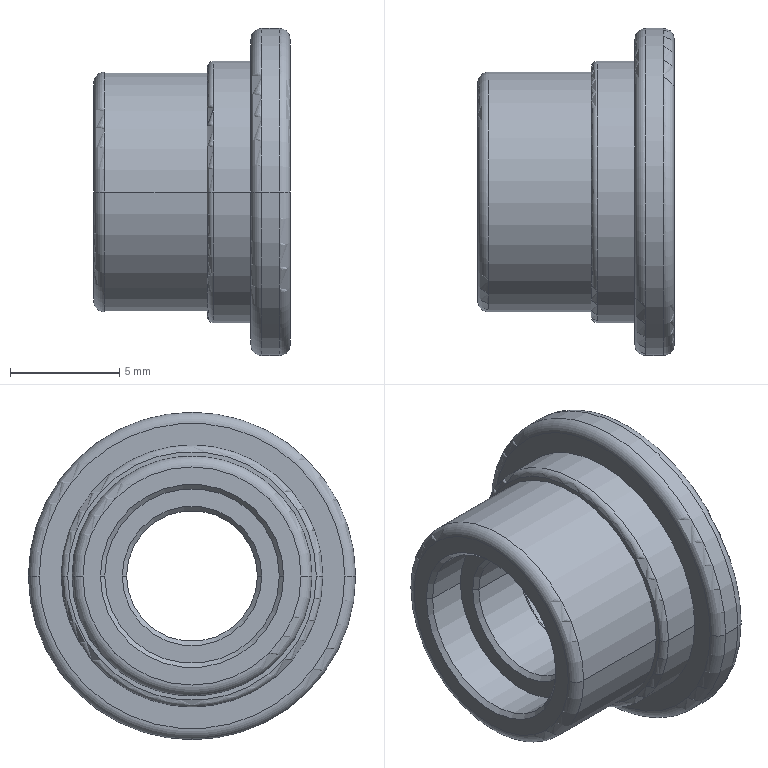Component | SolidWorks | 18MTOSC80BatteryCellCornerFoldingRollerAssembly-1_18ZTJ-NVT-01-001-1 | 1 solid | 39 faces | box 9 x 15 x 15 mm | volume 586 mm3 | cylinder 14 | cone 10 | torus 8 | plane 7 | commonest cylinder face diameters 8 x4 10 x2 11 x2 12 x2 15 x2 6 x2 | material Black POM
build123d program:
from build123d import *

# Parameters (mm, degrees)
SKETCH2_R          = 3
CUT_EXTRUDE1_DEPTH = 14.91
SKETCH3_R          = 5
CUT_EXTRUDE2_DEPTH = 2
FILLET1_R          = 0.5
FILLET2_R          = 0.3
SKETCH4_R          = 4
CUT_EXTRUDE3_DEPTH = 2
CUT_EXTRUDE4_START = -2
SKETCH5_R          = 4
CUT_EXTRUDE4_DEPTH = 2
CHAMFER1_SIZE      = 0.2


with BuildPart() as part:
    # Sketch1 → Revolve1 (revolve)
    with BuildSketch(Plane(origin=(0, 0, 0), x_dir=(1, 0, 0), z_dir=(0, 1, 0)), mode=Mode.PRIVATE) as revolve1_sk:
        Polygon((0, 0), (0, -9), (5.5, -9), (5.5, -3.8), (6, -3.8), (6, -1.8), (7.5, -1.8), (7.5, 0), align=None)
    revolve(revolve1_sk.sketch.rotate(Axis((0, 0, 0), (0, 0, 1)), 180), axis=Axis((0, 0, 0), (0, 0, 1)))

    # Sketch2 → Cut-Extrude1 (cut, through all)
    with BuildSketch(Plane.XY.offset(9)):
        Circle(SKETCH2_R)
    extrude(amount=-CUT_EXTRUDE1_DEPTH, mode=Mode.SUBTRACT)

    # Sketch3 → Cut-Extrude2 (cut)
    with BuildSketch(Plane(origin=(0, 0, 0), x_dir=(-1, 0, 0), z_dir=(0, 0, -1))):
        Circle(SKETCH3_R)
    extrude(amount=-CUT_EXTRUDE2_DEPTH, mode=Mode.SUBTRACT)

    # Fillet1
    fillet1_edges = [part.edges().sort_by_distance(p)[0] for p in [
        (5.5, 0, 9),
        (7.5, 0, 1.8),
        (7.5, 0, 0),
    ]]
    fillet(fillet1_edges, radius=FILLET1_R)

    # Fillet2
    fillet2_edges = [part.edges().sort_by_distance(p)[0] for p in [
        (6, 0, 3.8),
    ]]
    fillet(fillet2_edges, radius=FILLET2_R)

    # Sketch4 → Cut-Extrude3 (cut)
    with BuildSketch(Plane(origin=(0, 0, 2), x_dir=(-1, 0, 0), z_dir=(0, 0, -1))):
        Circle(SKETCH4_R)
    extrude(amount=-CUT_EXTRUDE3_DEPTH, mode=Mode.SUBTRACT)

    # Sketch5 → Cut-Extrude4 (cut)
    with BuildSketch(Plane.XY.offset(9).offset(CUT_EXTRUDE4_START)):
        with Locations(Location((0, 0, 0), (0, 0, 180))):
            Circle(SKETCH5_R)
    extrude(amount=CUT_EXTRUDE4_DEPTH, mode=Mode.SUBTRACT)

    # Chamfer1
    chamfer1_edges = [part.edges().sort_by_distance(p)[0] for p in [
        (5, 0, 0),
        (4, 0, 2),
        (-3, 0, 4),
        (4, 0, 9),
        (-3, 0, 7),
    ]]
    chamfer(chamfer1_edges, length=CHAMFER1_SIZE)


solid = part.part

# Placed as in the assembly
solid = solid.moved(Location((16.9, -14.53, 131), (0, -90, 0)))
STEP:
#1=CARTESIAN_POINT('',(0.6575,-0.3752,5.157));
#2=VERTEX_POINT('',#1);
#3=CARTESIAN_POINT('',(0.6575,-0.7689,5.157));
#4=VERTEX_POINT('',#3);
#5=CARTESIAN_POINT('',(0.6575,-0.572,5.157));
#6=DIRECTION('',(1.,0.,0.));
#7=DIRECTION('',(0.,1.,0.));
#8=AXIS2_PLACEMENT_3D('',#5,#6,#7);
#9=CIRCLE('',#8,0.1969);
#10=EDGE_CURVE('',#2,#4,#9,.T.);
#11=ORIENTED_EDGE('',*,*,#10,.F.);
#12=CARTESIAN_POINT('',(0.6654,-0.3673,5.157));
#13=VERTEX_POINT('',#12);
#14=CARTESIAN_POINT('',(0.6575,-0.3752,5.157));
#15=DIRECTION('',(0.7071,0.7071,-0.));
#16=VECTOR('',#15,39.37);
#17=LINE('',#14,#16);
#18=EDGE_CURVE('',#2,#13,#17,.T.);
#19=ORIENTED_EDGE('',*,*,#18,.T.);
#20=CARTESIAN_POINT('',(0.6654,-0.7768,5.157));
#21=VERTEX_POINT('',#20);
#22=CARTESIAN_POINT('',(0.6654,-0.572,5.157));
#23=DIRECTION('',(-1.,-0.,-0.));
#24=DIRECTION('',(0.,1.,0.));
#25=AXIS2_PLACEMENT_3D('',#22,#23,#24);
#26=CIRCLE('',#25,0.2047);
#27=EDGE_CURVE('',#21,#13,#26,.T.);
#28=ORIENTED_EDGE('',*,*,#27,.F.);
#29=CARTESIAN_POINT('',(0.6575,-0.7689,5.157));
#30=DIRECTION('',(0.7071,-0.7071,0.));
#31=VECTOR('',#30,39.37);
#32=LINE('',#29,#31);
#33=EDGE_CURVE('',#4,#21,#32,.T.);
#34=ORIENTED_EDGE('',*,*,#33,.F.);
#35=EDGE_LOOP('',(#11,#19,#28,#34));
#36=FACE_OUTER_BOUND('',#35,.T.);
#37=CARTESIAN_POINT('',(0.6575,-0.572,5.157));
#38=DIRECTION('',(1.,0.,0.));
#39=DIRECTION('',(0.,-1.,0.));
#40=AXIS2_PLACEMENT_3D('',#37,#38,#39);
#41=CONICAL_SURFACE('',#40,0.1969,0.7854);
#42=ADVANCED_FACE('',(#36),#41,.F.);
#43=CARTESIAN_POINT('',(0.5788,-0.4146,5.157));
#44=VERTEX_POINT('',#43);
#45=CARTESIAN_POINT('',(0.5788,-0.7295,5.157));
#46=VERTEX_POINT('',#45);
#47=CARTESIAN_POINT('',(0.5788,-0.572,5.157));
#48=DIRECTION('',(1.,0.,0.));
#49=DIRECTION('',(0.,-1.,0.));
#50=AXIS2_PLACEMENT_3D('',#47,#48,#49);
#51=CIRCLE('',#50,0.1575);
#52=EDGE_CURVE('',#44,#46,#51,.T.);
#53=ORIENTED_EDGE('',*,*,#52,.F.);
#54=CARTESIAN_POINT('',(0.5866,-0.4067,5.157));
#55=VERTEX_POINT('',#54);
#56=CARTESIAN_POINT('',(0.5788,-0.4146,5.157));
#57=DIRECTION('',(0.7071,0.7071,-0.));
#58=VECTOR('',#57,39.37);
#59=LINE('',#56,#58);
#60=EDGE_CURVE('',#44,#55,#59,.T.);
#61=ORIENTED_EDGE('',*,*,#60,.T.);
#62=CARTESIAN_POINT('',(0.5866,-0.7374,5.157));
#63=VERTEX_POINT('',#62);
#64=CARTESIAN_POINT('',(0.5866,-0.572,5.157));
#65=DIRECTION('',(-1.,-0.,-0.));
#66=DIRECTION('',(0.,-1.,0.));
#67=AXIS2_PLACEMENT_3D('',#64,#65,#66);
#68=CIRCLE('',#67,0.1654);
#69=EDGE_CURVE('',#63,#55,#68,.T.);
#70=ORIENTED_EDGE('',*,*,#69,.F.);
#71=CARTESIAN_POINT('',(0.5788,-0.7295,5.157));
#72=DIRECTION('',(0.7071,-0.7071,0.));
#73=VECTOR('',#72,39.37);
#74=LINE('',#71,#73);
#75=EDGE_CURVE('',#46,#63,#74,.T.);
#76=ORIENTED_EDGE('',*,*,#75,.F.);
#77=EDGE_LOOP('',(#53,#61,#70,#76));
#78=FACE_OUTER_BOUND('',#77,.T.);
#79=CARTESIAN_POINT('',(0.5788,-0.572,5.157));
#80=DIRECTION('',(1.,0.,0.));
#81=DIRECTION('',(0.,-1.,0.));
#82=AXIS2_PLACEMENT_3D('',#79,#80,#81);
#83=CONICAL_SURFACE('',#82,0.1575,0.7854);
#84=ADVANCED_FACE('',(#78),#83,.F.);
#85=CARTESIAN_POINT('',(0.5,-0.4539,5.157));
#86=VERTEX_POINT('',#85);
#87=CARTESIAN_POINT('',(0.5,-0.6901,5.157));
#88=VERTEX_POINT('',#87);
#89=CARTESIAN_POINT('',(0.5,-0.572,5.157));
#90=DIRECTION('',(1.,0.,0.));
#91=DIRECTION('',(0.,-1.,0.));
#92=AXIS2_PLACEMENT_3D('',#89,#90,#91);
#93=CIRCLE('',#92,0.1181);
#94=EDGE_CURVE('',#86,#88,#93,.T.);
#95=ORIENTED_EDGE('',*,*,#94,.F.);
#96=CARTESIAN_POINT('',(0.5079,-0.4461,5.157));
#97=VERTEX_POINT('',#96);
#98=CARTESIAN_POINT('',(0.5079,-0.4461,5.157));
#99=DIRECTION('',(0.7071,0.7071,-0.));
#100=VECTOR('',#99,39.37);
#101=LINE('',#98,#100);
#102=EDGE_CURVE('',#86,#97,#101,.T.);
#103=ORIENTED_EDGE('',*,*,#102,.T.);
#104=CARTESIAN_POINT('',(0.5079,-0.698,5.157));
#105=VERTEX_POINT('',#104);
#106=CARTESIAN_POINT('',(0.5079,-0.572,5.157));
#107=DIRECTION('',(-1.,-0.,-0.));
#108=DIRECTION('',(0.,-1.,0.));
#109=AXIS2_PLACEMENT_3D('',#106,#107,#108);
#110=CIRCLE('',#109,0.126);
#111=EDGE_CURVE('',#105,#97,#110,.T.);
#112=ORIENTED_EDGE('',*,*,#111,.F.);
#113=CARTESIAN_POINT('',(0.5079,-0.698,5.157));
#114=DIRECTION('',(0.7071,-0.7071,0.));
#115=VECTOR('',#114,39.37);
#116=LINE('',#113,#115);
#117=EDGE_CURVE('',#88,#105,#116,.T.);
#118=ORIENTED_EDGE('',*,*,#117,.F.);
#119=EDGE_LOOP('',(#95,#103,#112,#118));
#120=FACE_OUTER_BOUND('',#119,.T.);
#121=CARTESIAN_POINT('',(0.5079,-0.572,5.157));
#122=DIRECTION('',(1.,0.,0.));
#123=DIRECTION('',(0.,-1.,0.));
#124=AXIS2_PLACEMENT_3D('',#121,#122,#123);
#125=CONICAL_SURFACE('',#124,0.126,0.7854);
#126=ADVANCED_FACE('',(#120),#125,.F.);
#127=CARTESIAN_POINT('',(0.3977,-0.6901,5.157));
#128=VERTEX_POINT('',#127);
#129=CARTESIAN_POINT('',(0.3977,-0.4539,5.157));
#130=VERTEX_POINT('',#129);
#131=CARTESIAN_POINT('',(0.3977,-0.572,5.157));
#132=DIRECTION('',(-1.,-0.,-0.));
#133=DIRECTION('',(0.,1.,0.));
#134=AXIS2_PLACEMENT_3D('',#131,#132,#133);
#135=CIRCLE('',#134,0.1181);
#136=EDGE_CURVE('',#128,#130,#135,.T.);
#137=ORIENTED_EDGE('',*,*,#136,.F.);
#138=CARTESIAN_POINT('',(0.3898,-0.698,5.157));
#139=VERTEX_POINT('',#138);
#140=CARTESIAN_POINT('',(0.3898,-0.698,5.157));
#141=DIRECTION('',(-0.7071,-0.7071,-0.));
#142=VECTOR('',#141,39.37);
#143=LINE('',#140,#142);
#144=EDGE_CURVE('',#128,#139,#143,.T.);
#145=ORIENTED_EDGE('',*,*,#144,.T.);
#146=CARTESIAN_POINT('',(0.3898,-0.4461,5.157));
#147=VERTEX_POINT('',#146);
#148=CARTESIAN_POINT('',(0.3898,-0.572,5.157));
#149=DIRECTION('',(1.,0.,0.));
#150=DIRECTION('',(0.,1.,0.));
#151=AXIS2_PLACEMENT_3D('',#148,#149,#150);
#152=CIRCLE('',#151,0.126);
#153=EDGE_CURVE('',#147,#139,#152,.T.);
#154=ORIENTED_EDGE('',*,*,#153,.F.);
#155=CARTESIAN_POINT('',(0.3898,-0.4461,5.157));
#156=DIRECTION('',(-0.7071,0.7071,-0.));
#157=VECTOR('',#156,39.37);
#158=LINE('',#155,#157);
#159=EDGE_CURVE('',#130,#147,#158,.T.);
#160=ORIENTED_EDGE('',*,*,#159,.F.);
#161=EDGE_LOOP('',(#137,#145,#154,#160));
#162=FACE_OUTER_BOUND('',#161,.T.);
#163=CARTESIAN_POINT('',(0.3898,-0.572,5.157));
#164=DIRECTION('',(-1.,-0.,-0.));
#165=DIRECTION('',(0.,1.,0.));
#166=AXIS2_PLACEMENT_3D('',#163,#164,#165);
#167=CONICAL_SURFACE('',#166,0.126,0.7854);
#168=ADVANCED_FACE('',(#162),#167,.F.);
#169=CARTESIAN_POINT('',(0.3189,-0.7295,5.157));
#170=VERTEX_POINT('',#169);
#171=CARTESIAN_POINT('',(0.3189,-0.4146,5.157));
#172=VERTEX_POINT('',#171);
#173=CARTESIAN_POINT('',(0.3189,-0.572,5.157));
#174=DIRECTION('',(-1.,-0.,-0.));
#175=DIRECTION('',(0.,-1.,0.));
#176=AXIS2_PLACEMENT_3D('',#173,#174,#175);
#177=CIRCLE('',#176,0.1575);
#178=EDGE_CURVE('',#170,#172,#177,.T.);
#179=ORIENTED_EDGE('',*,*,#178,.F.);
#180=CARTESIAN_POINT('',(0.311,-0.7374,5.157));
#181=VERTEX_POINT('',#180);
#182=CARTESIAN_POINT('',(0.3189,-0.7295,5.157));
#183=DIRECTION('',(-0.7071,-0.7071,-0.));
#184=VECTOR('',#183,39.37);
#185=LINE('',#182,#184);
#186=EDGE_CURVE('',#170,#181,#185,.T.);
#187=ORIENTED_EDGE('',*,*,#186,.T.);
#188=CARTESIAN_POINT('',(0.311,-0.4067,5.157));
#189=VERTEX_POINT('',#188);
#190=CARTESIAN_POINT('',(0.311,-0.572,5.157));
#191=DIRECTION('',(1.,0.,0.));
#192=DIRECTION('',(0.,-1.,0.));
#193=AXIS2_PLACEMENT_3D('',#190,#191,#192);
#194=CIRCLE('',#193,0.1654);
#195=EDGE_CURVE('',#189,#181,#194,.T.);
#196=ORIENTED_EDGE('',*,*,#195,.F.);
#197=CARTESIAN_POINT('',(0.3189,-0.4146,5.157));
#198=DIRECTION('',(-0.7071,0.7071,-0.));
#199=VECTOR('',#198,39.37);
#200=LINE('',#197,#199);
#201=EDGE_CURVE('',#172,#189,#200,.T.);
#202=ORIENTED_EDGE('',*,*,#201,.F.);
#203=EDGE_LOOP('',(#179,#187,#196,#202));
#204=FACE_OUTER_BOUND('',#203,.T.);
#205=CARTESIAN_POINT('',(0.3189,-0.572,5.157));
#206=DIRECTION('',(-1.,-0.,-0.));
#207=DIRECTION('',(0.,1.,0.));
#208=AXIS2_PLACEMENT_3D('',#205,#206,#207);
#209=CONICAL_SURFACE('',#208,0.1575,0.7854);
#210=ADVANCED_FACE('',(#204),#209,.F.);
#211=CARTESIAN_POINT('',(0.3898,-0.7295,5.157));
#212=VERTEX_POINT('',#211);
#213=CARTESIAN_POINT('',(0.3898,-0.4146,5.157));
#214=VERTEX_POINT('',#213);
#215=CARTESIAN_POINT('',(0.3898,-0.572,5.157));
#216=DIRECTION('',(-1.,-0.,-0.));
#217=DIRECTION('',(0.,1.,0.));
#218=AXIS2_PLACEMENT_3D('',#215,#216,#217);
#219=CIRCLE('',#218,0.1575);
#220=EDGE_CURVE('',#212,#214,#219,.T.);
#221=ORIENTED_EDGE('',*,*,#220,.F.);
#222=CARTESIAN_POINT('',(0.3898,-0.7295,5.157));
#223=DIRECTION('',(-1.,-0.,-0.));
#224=VECTOR('',#223,39.37);
#225=LINE('',#222,#224);
#226=EDGE_CURVE('',#212,#170,#225,.T.);
#227=ORIENTED_EDGE('',*,*,#226,.T.);
#228=ORIENTED_EDGE('',*,*,#178,.T.);
#229=CARTESIAN_POINT('',(0.3898,-0.4146,5.157));
#230=DIRECTION('',(-1.,-0.,-0.));
#231=VECTOR('',#230,39.37);
#232=LINE('',#229,#231);
#233=EDGE_CURVE('',#214,#172,#232,.T.);
#234=ORIENTED_EDGE('',*,*,#233,.F.);
#235=EDGE_LOOP('',(#221,#227,#228,#234));
#236=FACE_OUTER_BOUND('',#235,.T.);
#237=CARTESIAN_POINT('',(0.3898,-0.572,5.157));
#238=DIRECTION('',(-1.,-0.,-0.));
#239=DIRECTION('',(0.,1.,0.));
#240=AXIS2_PLACEMENT_3D('',#237,#238,#239);
#241=CYLINDRICAL_SURFACE('',#240,0.1575);
#242=ADVANCED_FACE('',(#236),#241,.F.);
#243=CARTESIAN_POINT('',(0.5079,-0.4146,5.157));
#244=VERTEX_POINT('',#243);
#245=CARTESIAN_POINT('',(0.5079,-0.7295,5.157));
#246=VERTEX_POINT('',#245);
#247=CARTESIAN_POINT('',(0.5079,-0.572,5.157));
#248=DIRECTION('',(1.,0.,0.));
#249=DIRECTION('',(0.,-1.,0.));
#250=AXIS2_PLACEMENT_3D('',#247,#248,#249);
#251=CIRCLE('',#250,0.1575);
#252=EDGE_CURVE('',#244,#246,#251,.T.);
#253=ORIENTED_EDGE('',*,*,#252,.F.);
#254=CARTESIAN_POINT('',(0.5079,-0.4146,5.157));
#255=DIRECTION('',(1.,0.,0.));
#256=VECTOR('',#255,39.37);
#257=LINE('',#254,#256);
#258=EDGE_CURVE('',#244,#44,#257,.T.);
#259=ORIENTED_EDGE('',*,*,#258,.T.);
#260=ORIENTED_EDGE('',*,*,#52,.T.);
#261=CARTESIAN_POINT('',(0.5079,-0.7295,5.157));
#262=DIRECTION('',(1.,0.,0.));
#263=VECTOR('',#262,39.37);
#264=LINE('',#261,#263);
#265=EDGE_CURVE('',#246,#46,#264,.T.);
#266=ORIENTED_EDGE('',*,*,#265,.F.);
#267=EDGE_LOOP('',(#253,#259,#260,#266));
#268=FACE_OUTER_BOUND('',#267,.T.);
#269=CARTESIAN_POINT('',(0.5079,-0.572,5.157));
#270=DIRECTION('',(1.,0.,0.));
#271=DIRECTION('',(0.,-1.,0.));
#272=AXIS2_PLACEMENT_3D('',#269,#270,#271);
#273=CYLINDRICAL_SURFACE('',#272,0.1575);
#274=ADVANCED_FACE('',(#268),#273,.F.);
#275=CARTESIAN_POINT('',(0.5158,-0.3476,5.157));
#276=VERTEX_POINT('',#275);
#277=CARTESIAN_POINT('',(0.5158,-0.7964,5.157));
#278=VERTEX_POINT('',#277);
#279=CARTESIAN_POINT('',(0.5158,-0.572,5.157));
#280=DIRECTION('',(-1.,-0.,-0.));
#281=DIRECTION('',(0.,-1.,0.));
#282=AXIS2_PLACEMENT_3D('',#279,#280,#281);
#283=CIRCLE('',#282,0.2244);
#284=EDGE_CURVE('',#276,#278,#283,.T.);
#285=ORIENTED_EDGE('',*,*,#284,.F.);
#286=CARTESIAN_POINT('',(0.5276,-0.3358,5.157));
#287=VERTEX_POINT('',#286);
#288=CARTESIAN_POINT('',(0.5276,-0.3476,5.157));
#289=DIRECTION('',(0.,-0.,-1.));
#290=DIRECTION('',(0.,1.,0.));
#291=AXIS2_PLACEMENT_3D('',#288,#289,#290);
#292=CIRCLE('',#291,0.01181);
#293=EDGE_CURVE('',#276,#287,#292,.T.);
#294=ORIENTED_EDGE('',*,*,#293,.T.);
#295=CARTESIAN_POINT('',(0.5276,-0.8083,5.157));
#296=VERTEX_POINT('',#295);
#297=CARTESIAN_POINT('',(0.5276,-0.572,5.157));
#298=DIRECTION('',(1.,0.,0.));
#299=DIRECTION('',(0.,-1.,0.));
#300=AXIS2_PLACEMENT_3D('',#297,#298,#299);
#301=CIRCLE('',#300,0.2362);
#302=EDGE_CURVE('',#296,#287,#301,.T.);
#303=ORIENTED_EDGE('',*,*,#302,.F.);
#304=CARTESIAN_POINT('',(0.5276,-0.7964,5.157));
#305=DIRECTION('',(-0.,0.,1.));
#306=DIRECTION('',(1.,0.,0.));
#307=AXIS2_PLACEMENT_3D('',#304,#305,#306);
#308=CIRCLE('',#307,0.01181);
#309=EDGE_CURVE('',#278,#296,#308,.T.);
#310=ORIENTED_EDGE('',*,*,#309,.F.);
#311=EDGE_LOOP('',(#285,#294,#303,#310));
#312=FACE_OUTER_BOUND('',#311,.T.);
#313=CARTESIAN_POINT('',(0.5276,-0.572,5.157));
#314=DIRECTION('',(1.,0.,0.));
#315=DIRECTION('',(0.,-1.,0.));
#316=AXIS2_PLACEMENT_3D('',#313,#314,#315);
#317=TOROIDAL_SURFACE('',#316,0.2244,0.01181);
#318=ADVANCED_FACE('',(#312),#317,.T.);
#319=CARTESIAN_POINT('',(0.5945,-0.2964,5.157));
#320=VERTEX_POINT('',#319);
#321=CARTESIAN_POINT('',(0.5945,-0.8476,5.157));
#322=VERTEX_POINT('',#321);
#323=CARTESIAN_POINT('',(0.5945,-0.572,5.157));
#324=DIRECTION('',(-1.,-0.,-0.));
#325=DIRECTION('',(0.,-1.,0.));
#326=AXIS2_PLACEMENT_3D('',#323,#324,#325);
#327=CIRCLE('',#326,0.2756);
#328=EDGE_CURVE('',#320,#322,#327,.T.);
#329=ORIENTED_EDGE('',*,*,#328,.F.);
#330=CARTESIAN_POINT('',(0.6142,-0.2768,5.157));
#331=VERTEX_POINT('',#330);
#332=CARTESIAN_POINT('',(0.6142,-0.2964,5.157));
#333=DIRECTION('',(0.,-0.,-1.));
#334=DIRECTION('',(0.,1.,0.));
#335=AXIS2_PLACEMENT_3D('',#332,#333,#334);
#336=CIRCLE('',#335,0.01969);
#337=EDGE_CURVE('',#320,#331,#336,.T.);
#338=ORIENTED_EDGE('',*,*,#337,.T.);
#339=CARTESIAN_POINT('',(0.6142,-0.8673,5.157));
#340=VERTEX_POINT('',#339);
#341=CARTESIAN_POINT('',(0.6142,-0.572,5.157));
#342=DIRECTION('',(1.,0.,0.));
#343=DIRECTION('',(0.,-1.,0.));
#344=AXIS2_PLACEMENT_3D('',#341,#342,#343);
#345=CIRCLE('',#344,0.2953);
#346=EDGE_CURVE('',#340,#331,#345,.T.);
#347=ORIENTED_EDGE('',*,*,#346,.F.);
#348=CARTESIAN_POINT('',(0.6142,-0.8476,5.157));
#349=DIRECTION('',(-0.,0.,1.));
#350=DIRECTION('',(1.,0.,0.));
#351=AXIS2_PLACEMENT_3D('',#348,#349,#350);
#352=CIRCLE('',#351,0.01969);
#353=EDGE_CURVE('',#322,#340,#352,.T.);
#354=ORIENTED_EDGE('',*,*,#353,.F.);
#355=EDGE_LOOP('',(#329,#338,#347,#354));
#356=FACE_OUTER_BOUND('',#355,.T.);
#357=CARTESIAN_POINT('',(0.6142,-0.572,5.157));
#358=DIRECTION('',(1.,0.,0.));
#359=DIRECTION('',(0.,-1.,0.));
#360=AXIS2_PLACEMENT_3D('',#357,#358,#359);
#361=TOROIDAL_SURFACE('',#360,0.2756,0.01969);
#362=ADVANCED_FACE('',(#356),#361,.T.);
#363=CARTESIAN_POINT('',(0.6654,-0.8476,5.157));
#364=VERTEX_POINT('',#363);
#365=CARTESIAN_POINT('',(0.6654,-0.2964,5.157));
#366=VERTEX_POINT('',#365);
#367=CARTESIAN_POINT('',(0.6654,-0.572,5.157));
#368=DIRECTION('',(1.,0.,0.));
#369=DIRECTION('',(0.,1.,0.));
#370=AXIS2_PLACEMENT_3D('',#367,#368,#369);
#371=CIRCLE('',#370,0.2756);
#372=EDGE_CURVE('',#364,#366,#371,.T.);
#373=ORIENTED_EDGE('',*,*,#372,.F.);
#374=CARTESIAN_POINT('',(0.6457,-0.8673,5.157));
#375=VERTEX_POINT('',#374);
#376=CARTESIAN_POINT('',(0.6457,-0.8476,5.157));
#377=DIRECTION('',(0.,0.,-1.));
#378=DIRECTION('',(0.,1.,0.));
#379=AXIS2_PLACEMENT_3D('',#376,#377,#378);
#380=CIRCLE('',#379,0.01969);
#381=EDGE_CURVE('',#364,#375,#380,.T.);
#382=ORIENTED_EDGE('',*,*,#381,.T.);
#383=CARTESIAN_POINT('',(0.6457,-0.2768,5.157));
#384=VERTEX_POINT('',#383);
#385=CARTESIAN_POINT('',(0.6457,-0.572,5.157));
#386=DIRECTION('',(-1.,-0.,-0.));
#387=DIRECTION('',(0.,1.,0.));
#388=AXIS2_PLACEMENT_3D('',#385,#386,#387);
#389=CIRCLE('',#388,0.2953);
#390=EDGE_CURVE('',#384,#375,#389,.T.);
#391=ORIENTED_EDGE('',*,*,#390,.F.);
#392=CARTESIAN_POINT('',(0.6457,-0.2964,5.157));
#393=DIRECTION('',(-0.,0.,1.));
#394=DIRECTION('',(1.,0.,0.));
#395=AXIS2_PLACEMENT_3D('',#392,#393,#394);
#396=CIRCLE('',#395,0.01969);
#397=EDGE_CURVE('',#366,#384,#396,.T.);
#398=ORIENTED_EDGE('',*,*,#397,.F.);
#399=EDGE_LOOP('',(#373,#382,#391,#398));
#400=FACE_OUTER_BOUND('',#399,.T.);
#401=CARTESIAN_POINT('',(0.6457,-0.572,5.157));
#402=DIRECTION('',(-1.,-0.,-0.));
#403=DIRECTION('',(-0.,1.,-0.));
#404=AXIS2_PLACEMENT_3D('',#401,#402,#403);
#405=TOROIDAL_SURFACE('',#404,0.2756,0.01969);
#406=ADVANCED_FACE('',(#400),#405,.T.);
#407=CARTESIAN_POINT('',(0.311,-0.3752,5.157));
#408=VERTEX_POINT('',#407);
#409=CARTESIAN_POINT('',(0.311,-0.7689,5.157));
#410=VERTEX_POINT('',#409);
#411=CARTESIAN_POINT('',(0.311,-0.572,5.157));
#412=DIRECTION('',(-1.,-0.,-0.));
#413=DIRECTION('',(0.,-1.,0.));
#414=AXIS2_PLACEMENT_3D('',#411,#412,#413);
#415=CIRCLE('',#414,0.1969);
#416=EDGE_CURVE('',#408,#410,#415,.T.);
#417=ORIENTED_EDGE('',*,*,#416,.F.);
#418=CARTESIAN_POINT('',(0.3307,-0.3555,5.157));
#419=VERTEX_POINT('',#418);
#420=CARTESIAN_POINT('',(0.3307,-0.3752,5.157));
#421=DIRECTION('',(0.,-0.,-1.));
#422=DIRECTION('',(0.,1.,0.));
#423=AXIS2_PLACEMENT_3D('',#420,#421,#422);
#424=CIRCLE('',#423,0.01969);
#425=EDGE_CURVE('',#408,#419,#424,.T.);
#426=ORIENTED_EDGE('',*,*,#425,.T.);
#427=CARTESIAN_POINT('',(0.3307,-0.7886,5.157));
#428=VERTEX_POINT('',#427);
#429=CARTESIAN_POINT('',(0.3307,-0.572,5.157));
#430=DIRECTION('',(1.,0.,0.));
#431=DIRECTION('',(0.,-1.,0.));
#432=AXIS2_PLACEMENT_3D('',#429,#430,#431);
#433=CIRCLE('',#432,0.2165);
#434=EDGE_CURVE('',#428,#419,#433,.T.);
#435=ORIENTED_EDGE('',*,*,#434,.F.);
#436=CARTESIAN_POINT('',(0.3307,-0.7689,5.157));
#437=DIRECTION('',(-0.,0.,1.));
#438=DIRECTION('',(1.,0.,0.));
#439=AXIS2_PLACEMENT_3D('',#436,#437,#438);
#440=CIRCLE('',#439,0.01969);
#441=EDGE_CURVE('',#410,#428,#440,.T.);
#442=ORIENTED_EDGE('',*,*,#441,.F.);
#443=EDGE_LOOP('',(#417,#426,#435,#442));
#444=FACE_OUTER_BOUND('',#443,.T.);
#445=CARTESIAN_POINT('',(0.3307,-0.572,5.157));
#446=DIRECTION('',(1.,0.,0.));
#447=DIRECTION('',(0.,-1.,0.));
#448=AXIS2_PLACEMENT_3D('',#445,#446,#447);
#449=TOROIDAL_SURFACE('',#448,0.1969,0.01969);
#450=ADVANCED_FACE('',(#444),#449,.T.);
#451=CARTESIAN_POINT('',(0.5866,-0.3752,5.157));
#452=VERTEX_POINT('',#451);
#453=CARTESIAN_POINT('',(0.5866,-0.7689,5.157));
#454=VERTEX_POINT('',#453);
#455=CARTESIAN_POINT('',(0.5866,-0.572,5.157));
#456=DIRECTION('',(1.,0.,0.));
#457=DIRECTION('',(0.,-1.,0.));
#458=AXIS2_PLACEMENT_3D('',#455,#456,#457);
#459=CIRCLE('',#458,0.1969);
#460=EDGE_CURVE('',#452,#454,#459,.T.);
#461=ORIENTED_EDGE('',*,*,#460,.F.);
#462=CARTESIAN_POINT('',(0.5866,-0.3752,5.157));
#463=DIRECTION('',(1.,0.,0.));
#464=VECTOR('',#463,39.37);
#465=LINE('',#462,#464);
#466=EDGE_CURVE('',#452,#2,#465,.T.);
#467=ORIENTED_EDGE('',*,*,#466,.T.);
#468=ORIENTED_EDGE('',*,*,#10,.T.);
#469=CARTESIAN_POINT('',(0.5866,-0.7689,5.157));
#470=DIRECTION('',(1.,0.,0.));
#471=VECTOR('',#470,39.37);
#472=LINE('',#469,#471);
#473=EDGE_CURVE('',#454,#4,#472,.T.);
#474=ORIENTED_EDGE('',*,*,#473,.F.);
#475=EDGE_LOOP('',(#461,#467,#468,#474));
#476=FACE_OUTER_BOUND('',#475,.T.);
#477=CARTESIAN_POINT('',(0.5866,-0.572,5.157));
#478=DIRECTION('',(1.,0.,0.));
#479=DIRECTION('',(0.,-1.,0.));
#480=AXIS2_PLACEMENT_3D('',#477,#478,#479);
#481=CYLINDRICAL_SURFACE('',#480,0.1969);
#482=ADVANCED_FACE('',(#476),#481,.F.);
#483=ORIENTED_EDGE('',*,*,#434,.T.);
#484=CARTESIAN_POINT('',(0.5158,-0.3555,5.157));
#485=VERTEX_POINT('',#484);
#486=CARTESIAN_POINT('',(0.6654,-0.3555,5.157));
#487=DIRECTION('',(1.,0.,0.));
#488=VECTOR('',#487,39.37);
#489=LINE('',#486,#488);
#490=EDGE_CURVE('',#419,#485,#489,.T.);
#491=ORIENTED_EDGE('',*,*,#490,.T.);
#492=CARTESIAN_POINT('',(0.5158,-0.7886,5.157));
#493=VERTEX_POINT('',#492);
#494=CARTESIAN_POINT('',(0.5158,-0.572,5.157));
#495=DIRECTION('',(1.,0.,0.));
#496=DIRECTION('',(0.,-1.,0.));
#497=AXIS2_PLACEMENT_3D('',#494,#495,#496);
#498=CIRCLE('',#497,0.2165);
#499=EDGE_CURVE('',#493,#485,#498,.T.);
#500=ORIENTED_EDGE('',*,*,#499,.F.);
#501=CARTESIAN_POINT('',(0.6654,-0.7886,5.157));
#502=DIRECTION('',(1.,0.,0.));
#503=VECTOR('',#502,39.37);
#504=LINE('',#501,#503);
#505=EDGE_CURVE('',#428,#493,#504,.T.);
#506=ORIENTED_EDGE('',*,*,#505,.F.);
#507=EDGE_LOOP('',(#483,#491,#500,#506));
#508=FACE_OUTER_BOUND('',#507,.T.);
#509=CARTESIAN_POINT('',(0.6654,-0.572,5.157));
#510=DIRECTION('',(1.,0.,0.));
#511=DIRECTION('',(0.,-1.,0.));
#512=AXIS2_PLACEMENT_3D('',#509,#510,#511);
#513=CYLINDRICAL_SURFACE('',#512,0.2165);
#514=ADVANCED_FACE('',(#508),#513,.T.);
#515=ORIENTED_EDGE('',*,*,#302,.T.);
#516=CARTESIAN_POINT('',(0.5945,-0.3358,5.157));
#517=VERTEX_POINT('',#516);
#518=CARTESIAN_POINT('',(0.6654,-0.3358,5.157));
#519=DIRECTION('',(1.,0.,0.));
#520=VECTOR('',#519,39.37);
#521=LINE('',#518,#520);
#522=EDGE_CURVE('',#287,#517,#521,.T.);
#523=ORIENTED_EDGE('',*,*,#522,.T.);
#524=CARTESIAN_POINT('',(0.5945,-0.8083,5.157));
#525=VERTEX_POINT('',#524);
#526=CARTESIAN_POINT('',(0.5945,-0.572,5.157));
#527=DIRECTION('',(1.,0.,0.));
#528=DIRECTION('',(0.,-1.,0.));
#529=AXIS2_PLACEMENT_3D('',#526,#527,#528);
#530=CIRCLE('',#529,0.2362);
#531=EDGE_CURVE('',#525,#517,#530,.T.);
#532=ORIENTED_EDGE('',*,*,#531,.F.);
#533=CARTESIAN_POINT('',(0.6654,-0.8083,5.157));
#534=DIRECTION('',(1.,0.,0.));
#535=VECTOR('',#534,39.37);
#536=LINE('',#533,#535);
#537=EDGE_CURVE('',#296,#525,#536,.T.);
#538=ORIENTED_EDGE('',*,*,#537,.F.);
#539=EDGE_LOOP('',(#515,#523,#532,#538));
#540=FACE_OUTER_BOUND('',#539,.T.);
#541=CARTESIAN_POINT('',(0.6654,-0.572,5.157));
#542=DIRECTION('',(1.,0.,0.));
#543=DIRECTION('',(0.,-1.,0.));
#544=AXIS2_PLACEMENT_3D('',#541,#542,#543);
#545=CYLINDRICAL_SURFACE('',#544,0.2362);
#546=ADVANCED_FACE('',(#540),#545,.T.);
#547=ORIENTED_EDGE('',*,*,#346,.T.);
#548=CARTESIAN_POINT('',(0.6654,-0.2768,5.157));
#549=DIRECTION('',(1.,0.,0.));
#550=VECTOR('',#549,39.37);
#551=LINE('',#548,#550);
#552=EDGE_CURVE('',#331,#384,#551,.T.);
#553=ORIENTED_EDGE('',*,*,#552,.T.);
#554=ORIENTED_EDGE('',*,*,#390,.T.);
#555=CARTESIAN_POINT('',(0.6654,-0.8673,5.157));
#556=DIRECTION('',(1.,0.,0.));
#557=VECTOR('',#556,39.37);
#558=LINE('',#555,#557);
#559=EDGE_CURVE('',#340,#375,#558,.T.);
#560=ORIENTED_EDGE('',*,*,#559,.F.);
#561=EDGE_LOOP('',(#547,#553,#554,#560));
#562=FACE_OUTER_BOUND('',#561,.T.);
#563=CARTESIAN_POINT('',(0.6654,-0.572,5.157));
#564=DIRECTION('',(1.,0.,0.));
#565=DIRECTION('',(0.,-1.,0.));
#566=AXIS2_PLACEMENT_3D('',#563,#564,#565);
#567=CYLINDRICAL_SURFACE('',#566,0.2953);
#568=ADVANCED_FACE('',(#562),#567,.T.);
#569=ORIENTED_EDGE('',*,*,#94,.T.);
#570=CARTESIAN_POINT('',(0.6654,-0.6901,5.157));
#571=DIRECTION('',(-1.,-0.,-0.));
#572=VECTOR('',#571,39.37);
#573=LINE('',#570,#572);
#574=EDGE_CURVE('',#88,#128,#573,.T.);
#575=ORIENTED_EDGE('',*,*,#574,.T.);
#576=ORIENTED_EDGE('',*,*,#136,.T.);
#577=CARTESIAN_POINT('',(0.6654,-0.4539,5.157));
#578=DIRECTION('',(-1.,-0.,-0.));
#579=VECTOR('',#578,39.37);
#580=LINE('',#577,#579);
#581=EDGE_CURVE('',#86,#130,#580,.T.);
#582=ORIENTED_EDGE('',*,*,#581,.F.);
#583=EDGE_LOOP('',(#569,#575,#576,#582));
#584=FACE_OUTER_BOUND('',#583,.T.);
#585=CARTESIAN_POINT('',(0.6654,-0.572,5.157));
#586=DIRECTION('',(-1.,-0.,-0.));
#587=DIRECTION('',(0.,1.,0.));
#588=AXIS2_PLACEMENT_3D('',#585,#586,#587);
#589=CYLINDRICAL_SURFACE('',#588,0.1181);
#590=ADVANCED_FACE('',(#584),#589,.F.);
#591=ORIENTED_EDGE('',*,*,#574,.F.);
#592=CARTESIAN_POINT('',(0.5,-0.572,5.157));
#593=DIRECTION('',(1.,0.,0.));
#594=DIRECTION('',(0.,-1.,0.));
#595=AXIS2_PLACEMENT_3D('',#592,#593,#594);
#596=CIRCLE('',#595,0.1181);
#597=EDGE_CURVE('',#88,#86,#596,.T.);
#598=ORIENTED_EDGE('',*,*,#597,.T.);
#599=ORIENTED_EDGE('',*,*,#581,.T.);
#600=CARTESIAN_POINT('',(0.3977,-0.572,5.157));
#601=DIRECTION('',(-1.,-0.,-0.));
#602=DIRECTION('',(0.,1.,0.));
#603=AXIS2_PLACEMENT_3D('',#600,#601,#602);
#604=CIRCLE('',#603,0.1181);
#605=EDGE_CURVE('',#130,#128,#604,.T.);
#606=ORIENTED_EDGE('',*,*,#605,.T.);
#607=EDGE_LOOP('',(#591,#598,#599,#606));
#608=FACE_OUTER_BOUND('',#607,.T.);
#609=CARTESIAN_POINT('',(0.6654,-0.572,5.157));
#610=DIRECTION('',(-1.,-0.,-0.));
#611=DIRECTION('',(0.,1.,0.));
#612=AXIS2_PLACEMENT_3D('',#609,#610,#611);
#613=CYLINDRICAL_SURFACE('',#612,0.1181);
#614=ADVANCED_FACE('',(#608),#613,.F.);
#615=ORIENTED_EDGE('',*,*,#27,.T.);
#616=CARTESIAN_POINT('',(0.6654,-0.572,5.157));
#617=DIRECTION('',(-1.,-0.,-0.));
#618=DIRECTION('',(0.,1.,0.));
#619=AXIS2_PLACEMENT_3D('',#616,#617,#618);
#620=CIRCLE('',#619,0.2047);
#621=EDGE_CURVE('',#13,#21,#620,.T.);
#622=ORIENTED_EDGE('',*,*,#621,.T.);
#623=EDGE_LOOP('',(#615,#622));
#624=FACE_BOUND('',#623,.T.);
#625=CARTESIAN_POINT('',(0.6654,-0.572,5.157));
#626=DIRECTION('',(1.,0.,0.));
#627=DIRECTION('',(0.,1.,0.));
#628=AXIS2_PLACEMENT_3D('',#625,#626,#627);
#629=CIRCLE('',#628,0.2756);
#630=EDGE_CURVE('',#366,#364,#629,.T.);
#631=ORIENTED_EDGE('',*,*,#630,.T.);
#632=ORIENTED_EDGE('',*,*,#372,.T.);
#633=EDGE_LOOP('',(#631,#632));
#634=FACE_OUTER_BOUND('',#633,.T.);
#635=CARTESIAN_POINT('',(0.6654,-0.572,5.157));
#636=DIRECTION('',(-1.,-0.,-0.));
#637=DIRECTION('',(-0.,1.,-0.));
#638=AXIS2_PLACEMENT_3D('',#635,#636,#637);
#639=PLANE('',#638);
#640=ADVANCED_FACE('',(#624,#634),#639,.F.);
#641=ORIENTED_EDGE('',*,*,#552,.F.);
#642=CARTESIAN_POINT('',(0.6142,-0.572,5.157));
#643=DIRECTION('',(1.,0.,0.));
#644=DIRECTION('',(0.,-1.,0.));
#645=AXIS2_PLACEMENT_3D('',#642,#643,#644);
#646=CIRCLE('',#645,0.2953);
#647=EDGE_CURVE('',#331,#340,#646,.T.);
#648=ORIENTED_EDGE('',*,*,#647,.T.);
#649=ORIENTED_EDGE('',*,*,#559,.T.);
#650=CARTESIAN_POINT('',(0.6457,-0.572,5.157));
#651=DIRECTION('',(-1.,-0.,-0.));
#652=DIRECTION('',(0.,1.,0.));
#653=AXIS2_PLACEMENT_3D('',#650,#651,#652);
#654=CIRCLE('',#653,0.2953);
#655=EDGE_CURVE('',#375,#384,#654,.T.);
#656=ORIENTED_EDGE('',*,*,#655,.T.);
#657=EDGE_LOOP('',(#641,#648,#649,#656));
#658=FACE_OUTER_BOUND('',#657,.T.);
#659=CARTESIAN_POINT('',(0.6654,-0.572,5.157));
#660=DIRECTION('',(1.,0.,0.));
#661=DIRECTION('',(0.,-1.,0.));
#662=AXIS2_PLACEMENT_3D('',#659,#660,#661);
#663=CYLINDRICAL_SURFACE('',#662,0.2953);
#664=ADVANCED_FACE('',(#658),#663,.T.);
#665=CARTESIAN_POINT('',(0.5945,-0.572,5.157));
#666=DIRECTION('',(-1.,-0.,-0.));
#667=DIRECTION('',(0.,-1.,0.));
#668=AXIS2_PLACEMENT_3D('',#665,#666,#667);
#669=CIRCLE('',#668,0.2756);
#670=EDGE_CURVE('',#322,#320,#669,.T.);
#671=ORIENTED_EDGE('',*,*,#670,.T.);
#672=ORIENTED_EDGE('',*,*,#328,.T.);
#673=EDGE_LOOP('',(#671,#672));
#674=FACE_OUTER_BOUND('',#673,.T.);
#675=ORIENTED_EDGE('',*,*,#531,.T.);
#676=CARTESIAN_POINT('',(0.5945,-0.572,5.157));
#677=DIRECTION('',(1.,0.,0.));
#678=DIRECTION('',(0.,-1.,0.));
#679=AXIS2_PLACEMENT_3D('',#676,#677,#678);
#680=CIRCLE('',#679,0.2362);
#681=EDGE_CURVE('',#517,#525,#680,.T.);
#682=ORIENTED_EDGE('',*,*,#681,.T.);
#683=EDGE_LOOP('',(#675,#682));
#684=FACE_BOUND('',#683,.T.);
#685=CARTESIAN_POINT('',(0.5945,-0.2768,5.157));
#686=DIRECTION('',(1.,0.,0.));
#687=DIRECTION('',(0.,-1.,0.));
#688=AXIS2_PLACEMENT_3D('',#685,#686,#687);
#689=PLANE('',#688);
#690=ADVANCED_FACE('',(#674,#684),#689,.F.);
#691=ORIENTED_EDGE('',*,*,#522,.F.);
#692=CARTESIAN_POINT('',(0.5276,-0.572,5.157));
#693=DIRECTION('',(1.,0.,0.));
#694=DIRECTION('',(0.,-1.,0.));
#695=AXIS2_PLACEMENT_3D('',#692,#693,#694);
#696=CIRCLE('',#695,0.2362);
#697=EDGE_CURVE('',#287,#296,#696,.T.);
#698=ORIENTED_EDGE('',*,*,#697,.T.);
#699=ORIENTED_EDGE('',*,*,#537,.T.);
#700=ORIENTED_EDGE('',*,*,#681,.F.);
#701=EDGE_LOOP('',(#691,#698,#699,#700));
#702=FACE_OUTER_BOUND('',#701,.T.);
#703=CARTESIAN_POINT('',(0.6654,-0.572,5.157));
#704=DIRECTION('',(1.,0.,0.));
#705=DIRECTION('',(0.,-1.,0.));
#706=AXIS2_PLACEMENT_3D('',#703,#704,#705);
#707=CYLINDRICAL_SURFACE('',#706,0.2362);
#708=ADVANCED_FACE('',(#702),#707,.T.);
#709=CARTESIAN_POINT('',(0.5158,-0.572,5.157));
#710=DIRECTION('',(-1.,-0.,-0.));
#711=DIRECTION('',(0.,-1.,0.));
#712=AXIS2_PLACEMENT_3D('',#709,#710,#711);
#713=CIRCLE('',#712,0.2244);
#714=EDGE_CURVE('',#278,#276,#713,.T.);
#715=ORIENTED_EDGE('',*,*,#714,.T.);
#716=ORIENTED_EDGE('',*,*,#284,.T.);
#717=EDGE_LOOP('',(#715,#716));
#718=FACE_OUTER_BOUND('',#717,.T.);
#719=ORIENTED_EDGE('',*,*,#499,.T.);
#720=CARTESIAN_POINT('',(0.5158,-0.572,5.157));
#721=DIRECTION('',(1.,0.,0.));
#722=DIRECTION('',(0.,-1.,0.));
#723=AXIS2_PLACEMENT_3D('',#720,#721,#722);
#724=CIRCLE('',#723,0.2165);
#725=EDGE_CURVE('',#485,#493,#724,.T.);
#726=ORIENTED_EDGE('',*,*,#725,.T.);
#727=EDGE_LOOP('',(#719,#726));
#728=FACE_BOUND('',#727,.T.);
#729=CARTESIAN_POINT('',(0.5158,-0.3358,5.157));
#730=DIRECTION('',(1.,0.,0.));
#731=DIRECTION('',(0.,-1.,0.));
#732=AXIS2_PLACEMENT_3D('',#729,#730,#731);
#733=PLANE('',#732);
#734=ADVANCED_FACE('',(#718,#728),#733,.F.);
#735=ORIENTED_EDGE('',*,*,#490,.F.);
#736=CARTESIAN_POINT('',(0.3307,-0.572,5.157));
#737=DIRECTION('',(1.,0.,0.));
#738=DIRECTION('',(0.,-1.,0.));
#739=AXIS2_PLACEMENT_3D('',#736,#737,#738);
#740=CIRCLE('',#739,0.2165);
#741=EDGE_CURVE('',#419,#428,#740,.T.);
#742=ORIENTED_EDGE('',*,*,#741,.T.);
#743=ORIENTED_EDGE('',*,*,#505,.T.);
#744=ORIENTED_EDGE('',*,*,#725,.F.);
#745=EDGE_LOOP('',(#735,#742,#743,#744));
#746=FACE_OUTER_BOUND('',#745,.T.);
#747=CARTESIAN_POINT('',(0.6654,-0.572,5.157));
#748=DIRECTION('',(1.,0.,0.));
#749=DIRECTION('',(0.,-1.,0.));
#750=AXIS2_PLACEMENT_3D('',#747,#748,#749);
#751=CYLINDRICAL_SURFACE('',#750,0.2165);
#752=ADVANCED_FACE('',(#746),#751,.T.);
#753=ORIENTED_EDGE('',*,*,#195,.T.);
#754=CARTESIAN_POINT('',(0.311,-0.572,5.157));
#755=DIRECTION('',(1.,0.,0.));
#756=DIRECTION('',(0.,-1.,0.));
#757=AXIS2_PLACEMENT_3D('',#754,#755,#756);
#758=CIRCLE('',#757,0.1654);
#759=EDGE_CURVE('',#181,#189,#758,.T.);
#760=ORIENTED_EDGE('',*,*,#759,.T.);
#761=EDGE_LOOP('',(#753,#760));
#762=FACE_BOUND('',#761,.T.);
#763=CARTESIAN_POINT('',(0.311,-0.572,5.157));
#764=DIRECTION('',(-1.,-0.,-0.));
#765=DIRECTION('',(0.,-1.,0.));
#766=AXIS2_PLACEMENT_3D('',#763,#764,#765);
#767=CIRCLE('',#766,0.1969);
#768=EDGE_CURVE('',#410,#408,#767,.T.);
#769=ORIENTED_EDGE('',*,*,#768,.T.);
#770=ORIENTED_EDGE('',*,*,#416,.T.);
#771=EDGE_LOOP('',(#769,#770));
#772=FACE_OUTER_BOUND('',#771,.T.);
#773=CARTESIAN_POINT('',(0.311,-0.3555,5.157));
#774=DIRECTION('',(1.,0.,0.));
#775=DIRECTION('',(0.,-1.,0.));
#776=AXIS2_PLACEMENT_3D('',#773,#774,#775);
#777=PLANE('',#776);
#778=ADVANCED_FACE('',(#762,#772),#777,.F.);
#779=ORIENTED_EDGE('',*,*,#69,.T.);
#780=CARTESIAN_POINT('',(0.5866,-0.572,5.157));
#781=DIRECTION('',(-1.,-0.,-0.));
#782=DIRECTION('',(0.,-1.,0.));
#783=AXIS2_PLACEMENT_3D('',#780,#781,#782);
#784=CIRCLE('',#783,0.1654);
#785=EDGE_CURVE('',#55,#63,#784,.T.);
#786=ORIENTED_EDGE('',*,*,#785,.T.);
#787=EDGE_LOOP('',(#779,#786));
#788=FACE_BOUND('',#787,.T.);
#789=CARTESIAN_POINT('',(0.5866,-0.572,5.157));
#790=DIRECTION('',(1.,0.,0.));
#791=DIRECTION('',(0.,-1.,0.));
#792=AXIS2_PLACEMENT_3D('',#789,#790,#791);
#793=CIRCLE('',#792,0.1969);
#794=EDGE_CURVE('',#454,#452,#793,.T.);
#795=ORIENTED_EDGE('',*,*,#794,.T.);
#796=ORIENTED_EDGE('',*,*,#460,.T.);
#797=EDGE_LOOP('',(#795,#796));
#798=FACE_OUTER_BOUND('',#797,.T.);
#799=CARTESIAN_POINT('',(0.5866,-0.572,5.157));
#800=DIRECTION('',(1.,0.,0.));
#801=DIRECTION('',(0.,-1.,0.));
#802=AXIS2_PLACEMENT_3D('',#799,#800,#801);
#803=PLANE('',#802);
#804=ADVANCED_FACE('',(#788,#798),#803,.T.);
#805=ORIENTED_EDGE('',*,*,#466,.F.);
#806=ORIENTED_EDGE('',*,*,#794,.F.);
#807=ORIENTED_EDGE('',*,*,#473,.T.);
#808=CARTESIAN_POINT('',(0.6575,-0.572,5.157));
#809=DIRECTION('',(1.,0.,0.));
#810=DIRECTION('',(0.,1.,0.));
#811=AXIS2_PLACEMENT_3D('',#808,#809,#810);
#812=CIRCLE('',#811,0.1969);
#813=EDGE_CURVE('',#4,#2,#812,.T.);
#814=ORIENTED_EDGE('',*,*,#813,.T.);
#815=EDGE_LOOP('',(#805,#806,#807,#814));
#816=FACE_OUTER_BOUND('',#815,.T.);
#817=CARTESIAN_POINT('',(0.5866,-0.572,5.157));
#818=DIRECTION('',(1.,0.,0.));
#819=DIRECTION('',(0.,-1.,0.));
#820=AXIS2_PLACEMENT_3D('',#817,#818,#819);
#821=CYLINDRICAL_SURFACE('',#820,0.1969);
#822=ADVANCED_FACE('',(#816),#821,.F.);
#823=ORIENTED_EDGE('',*,*,#425,.F.);
#824=ORIENTED_EDGE('',*,*,#768,.F.);
#825=ORIENTED_EDGE('',*,*,#441,.T.);
#826=ORIENTED_EDGE('',*,*,#741,.F.);
#827=EDGE_LOOP('',(#823,#824,#825,#826));
#828=FACE_OUTER_BOUND('',#827,.T.);
#829=CARTESIAN_POINT('',(0.3307,-0.572,5.157));
#830=DIRECTION('',(1.,0.,0.));
#831=DIRECTION('',(0.,-1.,0.));
#832=AXIS2_PLACEMENT_3D('',#829,#830,#831);
#833=TOROIDAL_SURFACE('',#832,0.1969,0.01969);
#834=ADVANCED_FACE('',(#828),#833,.T.);
#835=ORIENTED_EDGE('',*,*,#381,.F.);
#836=ORIENTED_EDGE('',*,*,#630,.F.);
#837=ORIENTED_EDGE('',*,*,#397,.T.);
#838=ORIENTED_EDGE('',*,*,#655,.F.);
#839=EDGE_LOOP('',(#835,#836,#837,#838));
#840=FACE_OUTER_BOUND('',#839,.T.);
#841=CARTESIAN_POINT('',(0.6457,-0.572,5.157));
#842=DIRECTION('',(-1.,-0.,-0.));
#843=DIRECTION('',(-0.,1.,-0.));
#844=AXIS2_PLACEMENT_3D('',#841,#842,#843);
#845=TOROIDAL_SURFACE('',#844,0.2756,0.01969);
#846=ADVANCED_FACE('',(#840),#845,.T.);
#847=ORIENTED_EDGE('',*,*,#337,.F.);
#848=ORIENTED_EDGE('',*,*,#670,.F.);
#849=ORIENTED_EDGE('',*,*,#353,.T.);
#850=ORIENTED_EDGE('',*,*,#647,.F.);
#851=EDGE_LOOP('',(#847,#848,#849,#850));
#852=FACE_OUTER_BOUND('',#851,.T.);
#853=CARTESIAN_POINT('',(0.6142,-0.572,5.157));
#854=DIRECTION('',(1.,0.,0.));
#855=DIRECTION('',(0.,-1.,0.));
#856=AXIS2_PLACEMENT_3D('',#853,#854,#855);
#857=TOROIDAL_SURFACE('',#856,0.2756,0.01969);
#858=ADVANCED_FACE('',(#852),#857,.T.);
#859=ORIENTED_EDGE('',*,*,#293,.F.);
#860=ORIENTED_EDGE('',*,*,#714,.F.);
#861=ORIENTED_EDGE('',*,*,#309,.T.);
#862=ORIENTED_EDGE('',*,*,#697,.F.);
#863=EDGE_LOOP('',(#859,#860,#861,#862));
#864=FACE_OUTER_BOUND('',#863,.T.);
#865=CARTESIAN_POINT('',(0.5276,-0.572,5.157));
#866=DIRECTION('',(1.,0.,0.));
#867=DIRECTION('',(0.,-1.,0.));
#868=AXIS2_PLACEMENT_3D('',#865,#866,#867);
#869=TOROIDAL_SURFACE('',#868,0.2244,0.01181);
#870=ADVANCED_FACE('',(#864),#869,.T.);
#871=ORIENTED_EDGE('',*,*,#111,.T.);
#872=CARTESIAN_POINT('',(0.5079,-0.572,5.157));
#873=DIRECTION('',(-1.,-0.,-0.));
#874=DIRECTION('',(0.,-1.,0.));
#875=AXIS2_PLACEMENT_3D('',#872,#873,#874);
#876=CIRCLE('',#875,0.126);
#877=EDGE_CURVE('',#97,#105,#876,.T.);
#878=ORIENTED_EDGE('',*,*,#877,.T.);
#879=EDGE_LOOP('',(#871,#878));
#880=FACE_BOUND('',#879,.T.);
#881=CARTESIAN_POINT('',(0.5079,-0.572,5.157));
#882=DIRECTION('',(1.,0.,0.));
#883=DIRECTION('',(0.,-1.,0.));
#884=AXIS2_PLACEMENT_3D('',#881,#882,#883);
#885=CIRCLE('',#884,0.1575);
#886=EDGE_CURVE('',#246,#244,#885,.T.);
#887=ORIENTED_EDGE('',*,*,#886,.T.);
#888=ORIENTED_EDGE('',*,*,#252,.T.);
#889=EDGE_LOOP('',(#887,#888));
#890=FACE_OUTER_BOUND('',#889,.T.);
#891=CARTESIAN_POINT('',(0.5079,-0.572,5.157));
#892=DIRECTION('',(1.,0.,0.));
#893=DIRECTION('',(0.,-1.,0.));
#894=AXIS2_PLACEMENT_3D('',#891,#892,#893);
#895=PLANE('',#894);
#896=ADVANCED_FACE('',(#880,#890),#895,.T.);
#897=ORIENTED_EDGE('',*,*,#258,.F.);
#898=ORIENTED_EDGE('',*,*,#886,.F.);
#899=ORIENTED_EDGE('',*,*,#265,.T.);
#900=CARTESIAN_POINT('',(0.5788,-0.572,5.157));
#901=DIRECTION('',(1.,0.,0.));
#902=DIRECTION('',(0.,-1.,0.));
#903=AXIS2_PLACEMENT_3D('',#900,#901,#902);
#904=CIRCLE('',#903,0.1575);
#905=EDGE_CURVE('',#46,#44,#904,.T.);
#906=ORIENTED_EDGE('',*,*,#905,.T.);
#907=EDGE_LOOP('',(#897,#898,#899,#906));
#908=FACE_OUTER_BOUND('',#907,.T.);
#909=CARTESIAN_POINT('',(0.5079,-0.572,5.157));
#910=DIRECTION('',(1.,0.,0.));
#911=DIRECTION('',(0.,-1.,0.));
#912=AXIS2_PLACEMENT_3D('',#909,#910,#911);
#913=CYLINDRICAL_SURFACE('',#912,0.1575);
#914=ADVANCED_FACE('',(#908),#913,.F.);
#915=ORIENTED_EDGE('',*,*,#153,.T.);
#916=CARTESIAN_POINT('',(0.3898,-0.572,5.157));
#917=DIRECTION('',(1.,0.,0.));
#918=DIRECTION('',(0.,1.,0.));
#919=AXIS2_PLACEMENT_3D('',#916,#917,#918);
#920=CIRCLE('',#919,0.126);
#921=EDGE_CURVE('',#139,#147,#920,.T.);
#922=ORIENTED_EDGE('',*,*,#921,.T.);
#923=EDGE_LOOP('',(#915,#922));
#924=FACE_BOUND('',#923,.T.);
#925=CARTESIAN_POINT('',(0.3898,-0.572,5.157));
#926=DIRECTION('',(-1.,-0.,-0.));
#927=DIRECTION('',(0.,1.,0.));
#928=AXIS2_PLACEMENT_3D('',#925,#926,#927);
#929=CIRCLE('',#928,0.1575);
#930=EDGE_CURVE('',#214,#212,#929,.T.);
#931=ORIENTED_EDGE('',*,*,#930,.T.);
#932=ORIENTED_EDGE('',*,*,#220,.T.);
#933=EDGE_LOOP('',(#931,#932));
#934=FACE_OUTER_BOUND('',#933,.T.);
#935=CARTESIAN_POINT('',(0.3898,-0.572,5.157));
#936=DIRECTION('',(-1.,-0.,-0.));
#937=DIRECTION('',(-0.,1.,-0.));
#938=AXIS2_PLACEMENT_3D('',#935,#936,#937);
#939=PLANE('',#938);
#940=ADVANCED_FACE('',(#924,#934),#939,.T.);
#941=ORIENTED_EDGE('',*,*,#226,.F.);
#942=ORIENTED_EDGE('',*,*,#930,.F.);
#943=ORIENTED_EDGE('',*,*,#233,.T.);
#944=CARTESIAN_POINT('',(0.3189,-0.572,5.157));
#945=DIRECTION('',(-1.,-0.,-0.));
#946=DIRECTION('',(0.,-1.,0.));
#947=AXIS2_PLACEMENT_3D('',#944,#945,#946);
#948=CIRCLE('',#947,0.1575);
#949=EDGE_CURVE('',#172,#170,#948,.T.);
#950=ORIENTED_EDGE('',*,*,#949,.T.);
#951=EDGE_LOOP('',(#941,#942,#943,#950));
#952=FACE_OUTER_BOUND('',#951,.T.);
#953=CARTESIAN_POINT('',(0.3898,-0.572,5.157));
#954=DIRECTION('',(-1.,-0.,-0.));
#955=DIRECTION('',(0.,1.,0.));
#956=AXIS2_PLACEMENT_3D('',#953,#954,#955);
#957=CYLINDRICAL_SURFACE('',#956,0.1575);
#958=ADVANCED_FACE('',(#952),#957,.F.);
#959=ORIENTED_EDGE('',*,*,#186,.F.);
#960=ORIENTED_EDGE('',*,*,#949,.F.);
#961=ORIENTED_EDGE('',*,*,#201,.T.);
#962=ORIENTED_EDGE('',*,*,#759,.F.);
#963=EDGE_LOOP('',(#959,#960,#961,#962));
#964=FACE_OUTER_BOUND('',#963,.T.);
#965=CARTESIAN_POINT('',(0.3189,-0.572,5.157));
#966=DIRECTION('',(-1.,-0.,-0.));
#967=DIRECTION('',(0.,1.,0.));
#968=AXIS2_PLACEMENT_3D('',#965,#966,#967);
#969=CONICAL_SURFACE('',#968,0.1575,0.7854);
#970=ADVANCED_FACE('',(#964),#969,.F.);
#971=ORIENTED_EDGE('',*,*,#144,.F.);
#972=ORIENTED_EDGE('',*,*,#605,.F.);
#973=ORIENTED_EDGE('',*,*,#159,.T.);
#974=ORIENTED_EDGE('',*,*,#921,.F.);
#975=EDGE_LOOP('',(#971,#972,#973,#974));
#976=FACE_OUTER_BOUND('',#975,.T.);
#977=CARTESIAN_POINT('',(0.3898,-0.572,5.157));
#978=DIRECTION('',(-1.,-0.,-0.));
#979=DIRECTION('',(0.,1.,0.));
#980=AXIS2_PLACEMENT_3D('',#977,#978,#979);
#981=CONICAL_SURFACE('',#980,0.126,0.7854);
#982=ADVANCED_FACE('',(#976),#981,.F.);
#983=ORIENTED_EDGE('',*,*,#102,.F.);
#984=ORIENTED_EDGE('',*,*,#597,.F.);
#985=ORIENTED_EDGE('',*,*,#117,.T.);
#986=ORIENTED_EDGE('',*,*,#877,.F.);
#987=EDGE_LOOP('',(#983,#984,#985,#986));
#988=FACE_OUTER_BOUND('',#987,.T.);
#989=CARTESIAN_POINT('',(0.5079,-0.572,5.157));
#990=DIRECTION('',(1.,0.,0.));
#991=DIRECTION('',(0.,-1.,0.));
#992=AXIS2_PLACEMENT_3D('',#989,#990,#991);
#993=CONICAL_SURFACE('',#992,0.126,0.7854);
#994=ADVANCED_FACE('',(#988),#993,.F.);
#995=ORIENTED_EDGE('',*,*,#60,.F.);
#996=ORIENTED_EDGE('',*,*,#905,.F.);
#997=ORIENTED_EDGE('',*,*,#75,.T.);
#998=ORIENTED_EDGE('',*,*,#785,.F.);
#999=EDGE_LOOP('',(#995,#996,#997,#998));
#1000=FACE_OUTER_BOUND('',#999,.T.);
#1001=CARTESIAN_POINT('',(0.5788,-0.572,5.157));
#1002=DIRECTION('',(1.,0.,0.));
#1003=DIRECTION('',(0.,-1.,0.));
#1004=AXIS2_PLACEMENT_3D('',#1001,#1002,#1003);
#1005=CONICAL_SURFACE('',#1004,0.1575,0.7854);
#1006=ADVANCED_FACE('',(#1000),#1005,.F.);
#1007=ORIENTED_EDGE('',*,*,#18,.F.);
#1008=ORIENTED_EDGE('',*,*,#813,.F.);
#1009=ORIENTED_EDGE('',*,*,#33,.T.);
#1010=ORIENTED_EDGE('',*,*,#621,.F.);
#1011=EDGE_LOOP('',(#1007,#1008,#1009,#1010));
#1012=FACE_OUTER_BOUND('',#1011,.T.);
#1013=CARTESIAN_POINT('',(0.6575,-0.572,5.157));
#1014=DIRECTION('',(1.,0.,0.));
#1015=DIRECTION('',(0.,-1.,0.));
#1016=AXIS2_PLACEMENT_3D('',#1013,#1014,#1015);
#1017=CONICAL_SURFACE('',#1016,0.1969,0.7854);
#1018=ADVANCED_FACE('',(#1012),#1017,.F.);
#1019=CLOSED_SHELL('',(#42,#84,#126,#168,#210,#242,#274,#318,#362,#406,#450,#482,#514,#546,#568,#590,#614,#640,#664,#690,#708,#734,#752,#778,#804,#822,#834,#846,#858,#870,#896,#914,#940,#958,#970,#982,#994,#1006,#1018));
#1020=MANIFOLD_SOLID_BREP('',#1019);
#1021=CARTESIAN_POINT('',(0.,0.,0.));
#1022=DIRECTION('',(0.,0.,1.));
#1023=DIRECTION('',(1.,0.,0.));
#1024=AXIS2_PLACEMENT_3D('',#1021,#1022,#1023);
#1025=(LENGTH_UNIT()NAMED_UNIT(*)SI_UNIT($,.METRE.));
#1026=LENGTH_MEASURE_WITH_UNIT(LENGTH_MEASURE(0.0254),#1025);
#1027=DIMENSIONAL_EXPONENTS(1.,0.,0.,0.,0.,0.,0.);
#1028=(CONVERSION_BASED_UNIT('',#1026)LENGTH_UNIT()NAMED_UNIT(#1027));
#1029=UNCERTAINTY_MEASURE_WITH_UNIT(LENGTH_MEASURE(0.00001),#1028,'','');
#1030=(NAMED_UNIT(*)PLANE_ANGLE_UNIT()SI_UNIT($,.RADIAN.));
#1031=(NAMED_UNIT(*)SI_UNIT($,.STERADIAN.)SOLID_ANGLE_UNIT());
#1032=(GEOMETRIC_REPRESENTATION_CONTEXT(3)GLOBAL_UNCERTAINTY_ASSIGNED_CONTEXT((#1029))GLOBAL_UNIT_ASSIGNED_CONTEXT((#1028,#1030,#1031))REPRESENTATION_CONTEXT('',''));
#1033=ADVANCED_BREP_SHAPE_REPRESENTATION('',(#1020,#1024),#1032);
#1034=COLOUR_RGB('',0.7922,0.8196,0.9333);
#1035=FILL_AREA_STYLE_COLOUR('',#1034);
#1036=FILL_AREA_STYLE('',(#1035));
#1037=SURFACE_STYLE_FILL_AREA(#1036);
#1038=SURFACE_SIDE_STYLE('',(#1037));
#1039=SURFACE_STYLE_USAGE(.BOTH.,#1038);
#1040=PRESENTATION_STYLE_ASSIGNMENT((#1039));
#1041=STYLED_ITEM('',(#1040),#1020);
#1042=(LENGTH_UNIT()NAMED_UNIT(*)SI_UNIT($,.METRE.));
#1043=LENGTH_MEASURE_WITH_UNIT(LENGTH_MEASURE(0.0254),#1042);
#1044=DIMENSIONAL_EXPONENTS(1.,0.,0.,0.,0.,0.,0.);
#1045=(CONVERSION_BASED_UNIT('',#1043)LENGTH_UNIT()NAMED_UNIT(#1044));
#1046=UNCERTAINTY_MEASURE_WITH_UNIT(LENGTH_MEASURE(0.00001),#1045,'','');
#1047=(NAMED_UNIT(*)PLANE_ANGLE_UNIT()SI_UNIT($,.RADIAN.));
#1048=(NAMED_UNIT(*)SI_UNIT($,.STERADIAN.)SOLID_ANGLE_UNIT());
#1049=(GEOMETRIC_REPRESENTATION_CONTEXT(3)GLOBAL_UNCERTAINTY_ASSIGNED_CONTEXT((#1046))GLOBAL_UNIT_ASSIGNED_CONTEXT((#1045,#1047,#1048))REPRESENTATION_CONTEXT('',''));
#1050=MECHANICAL_DESIGN_GEOMETRIC_PRESENTATION_REPRESENTATION('',(#1041),#1049);
#1051=PRESENTATION_LAYER_ASSIGNMENT('','',(#1041));